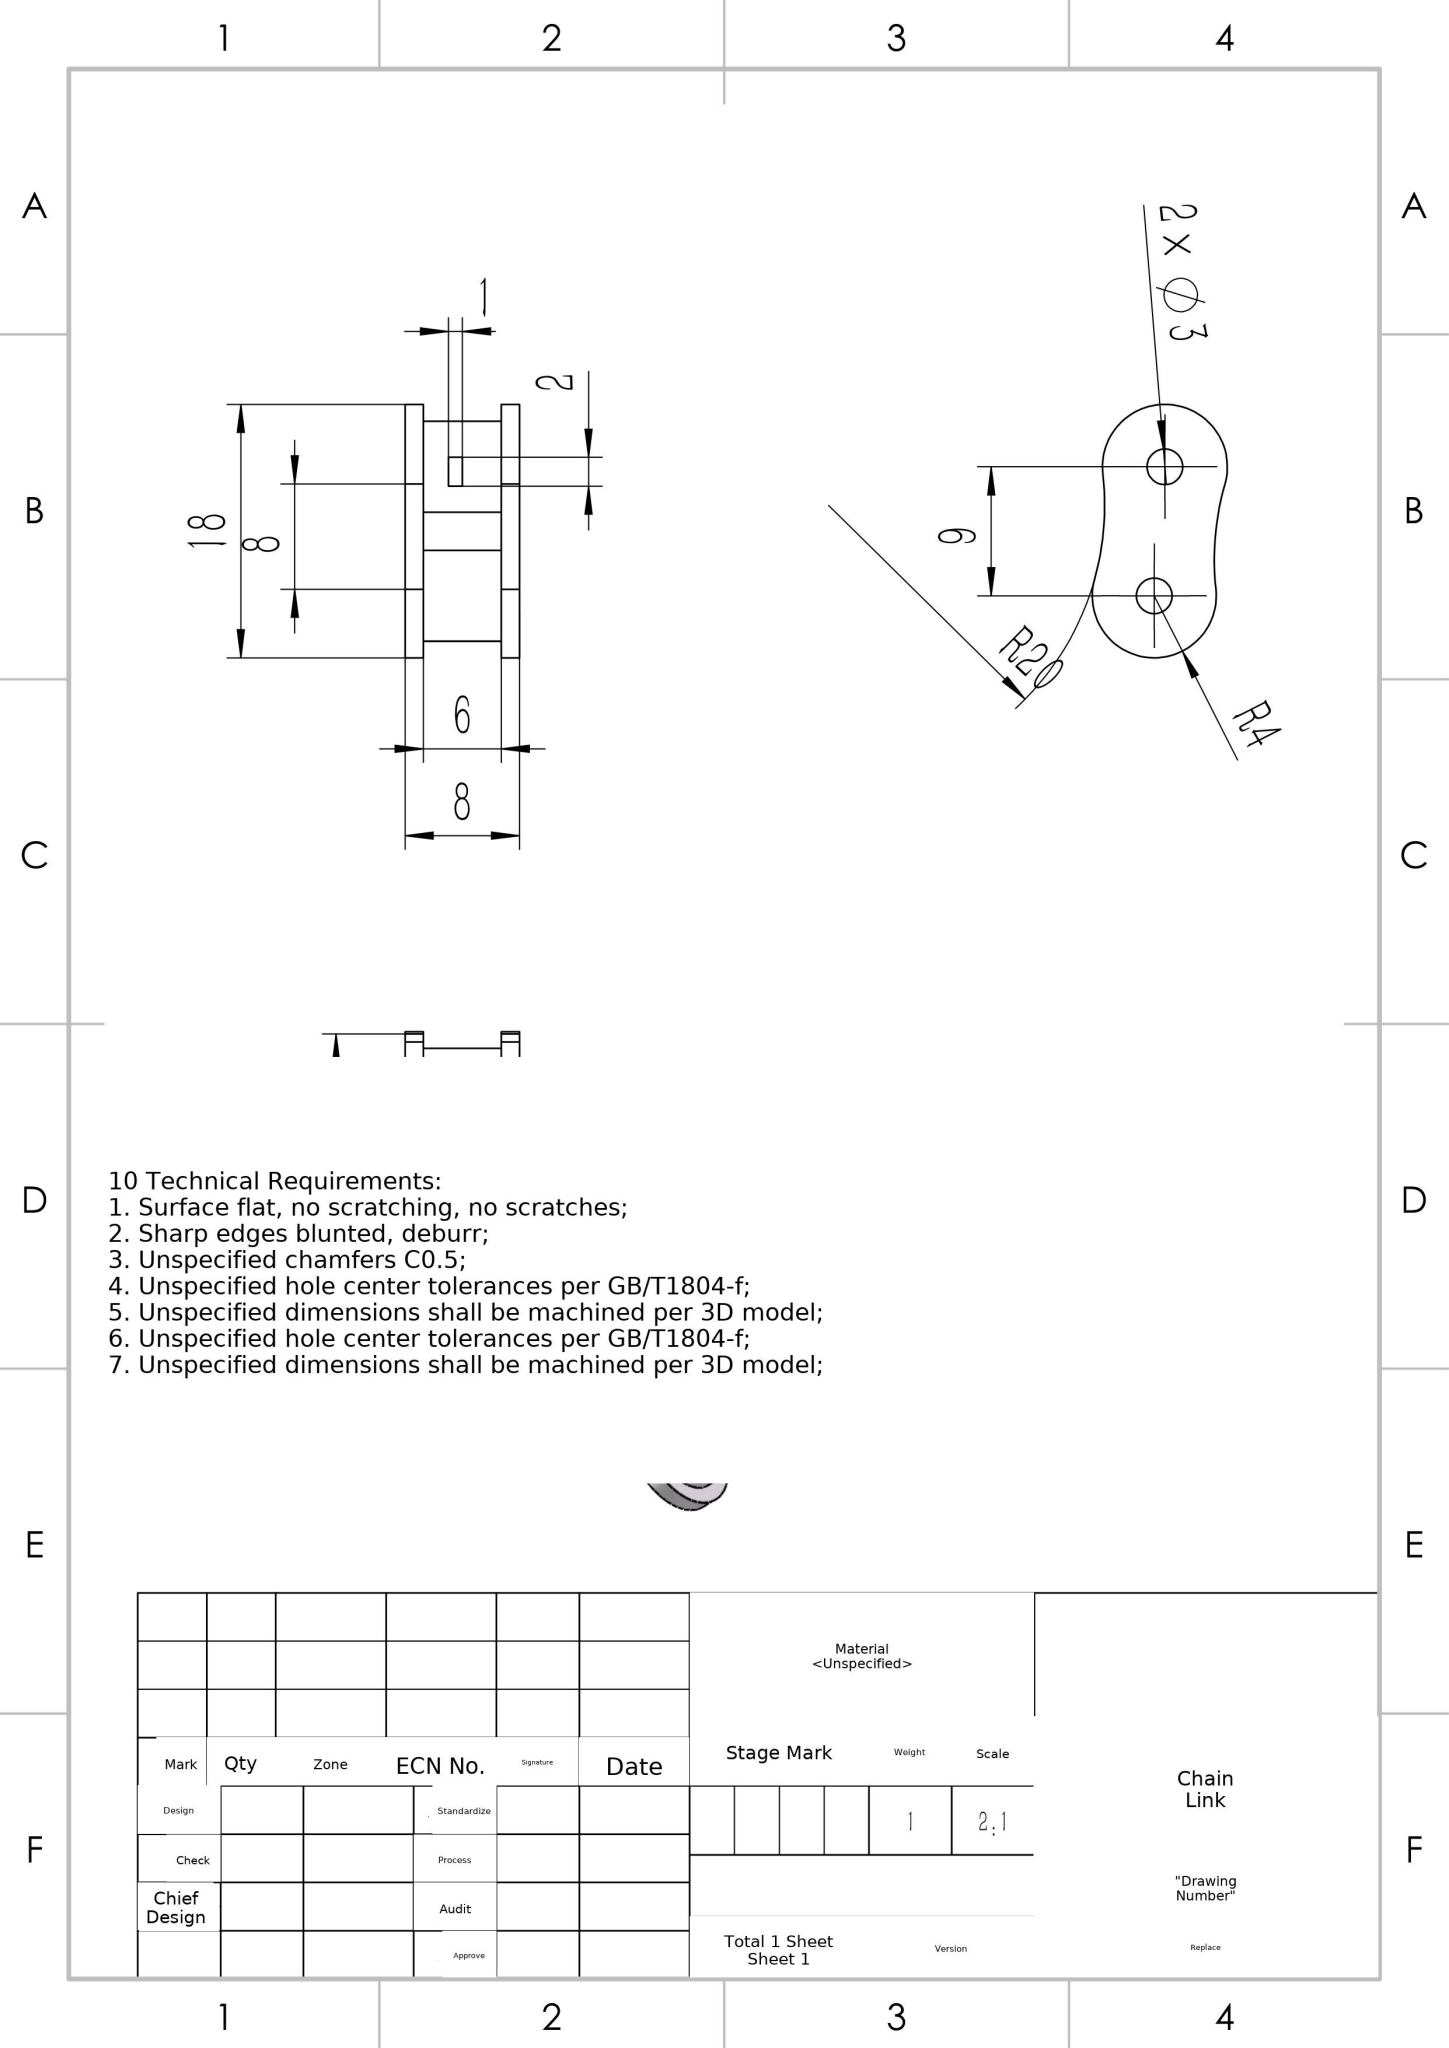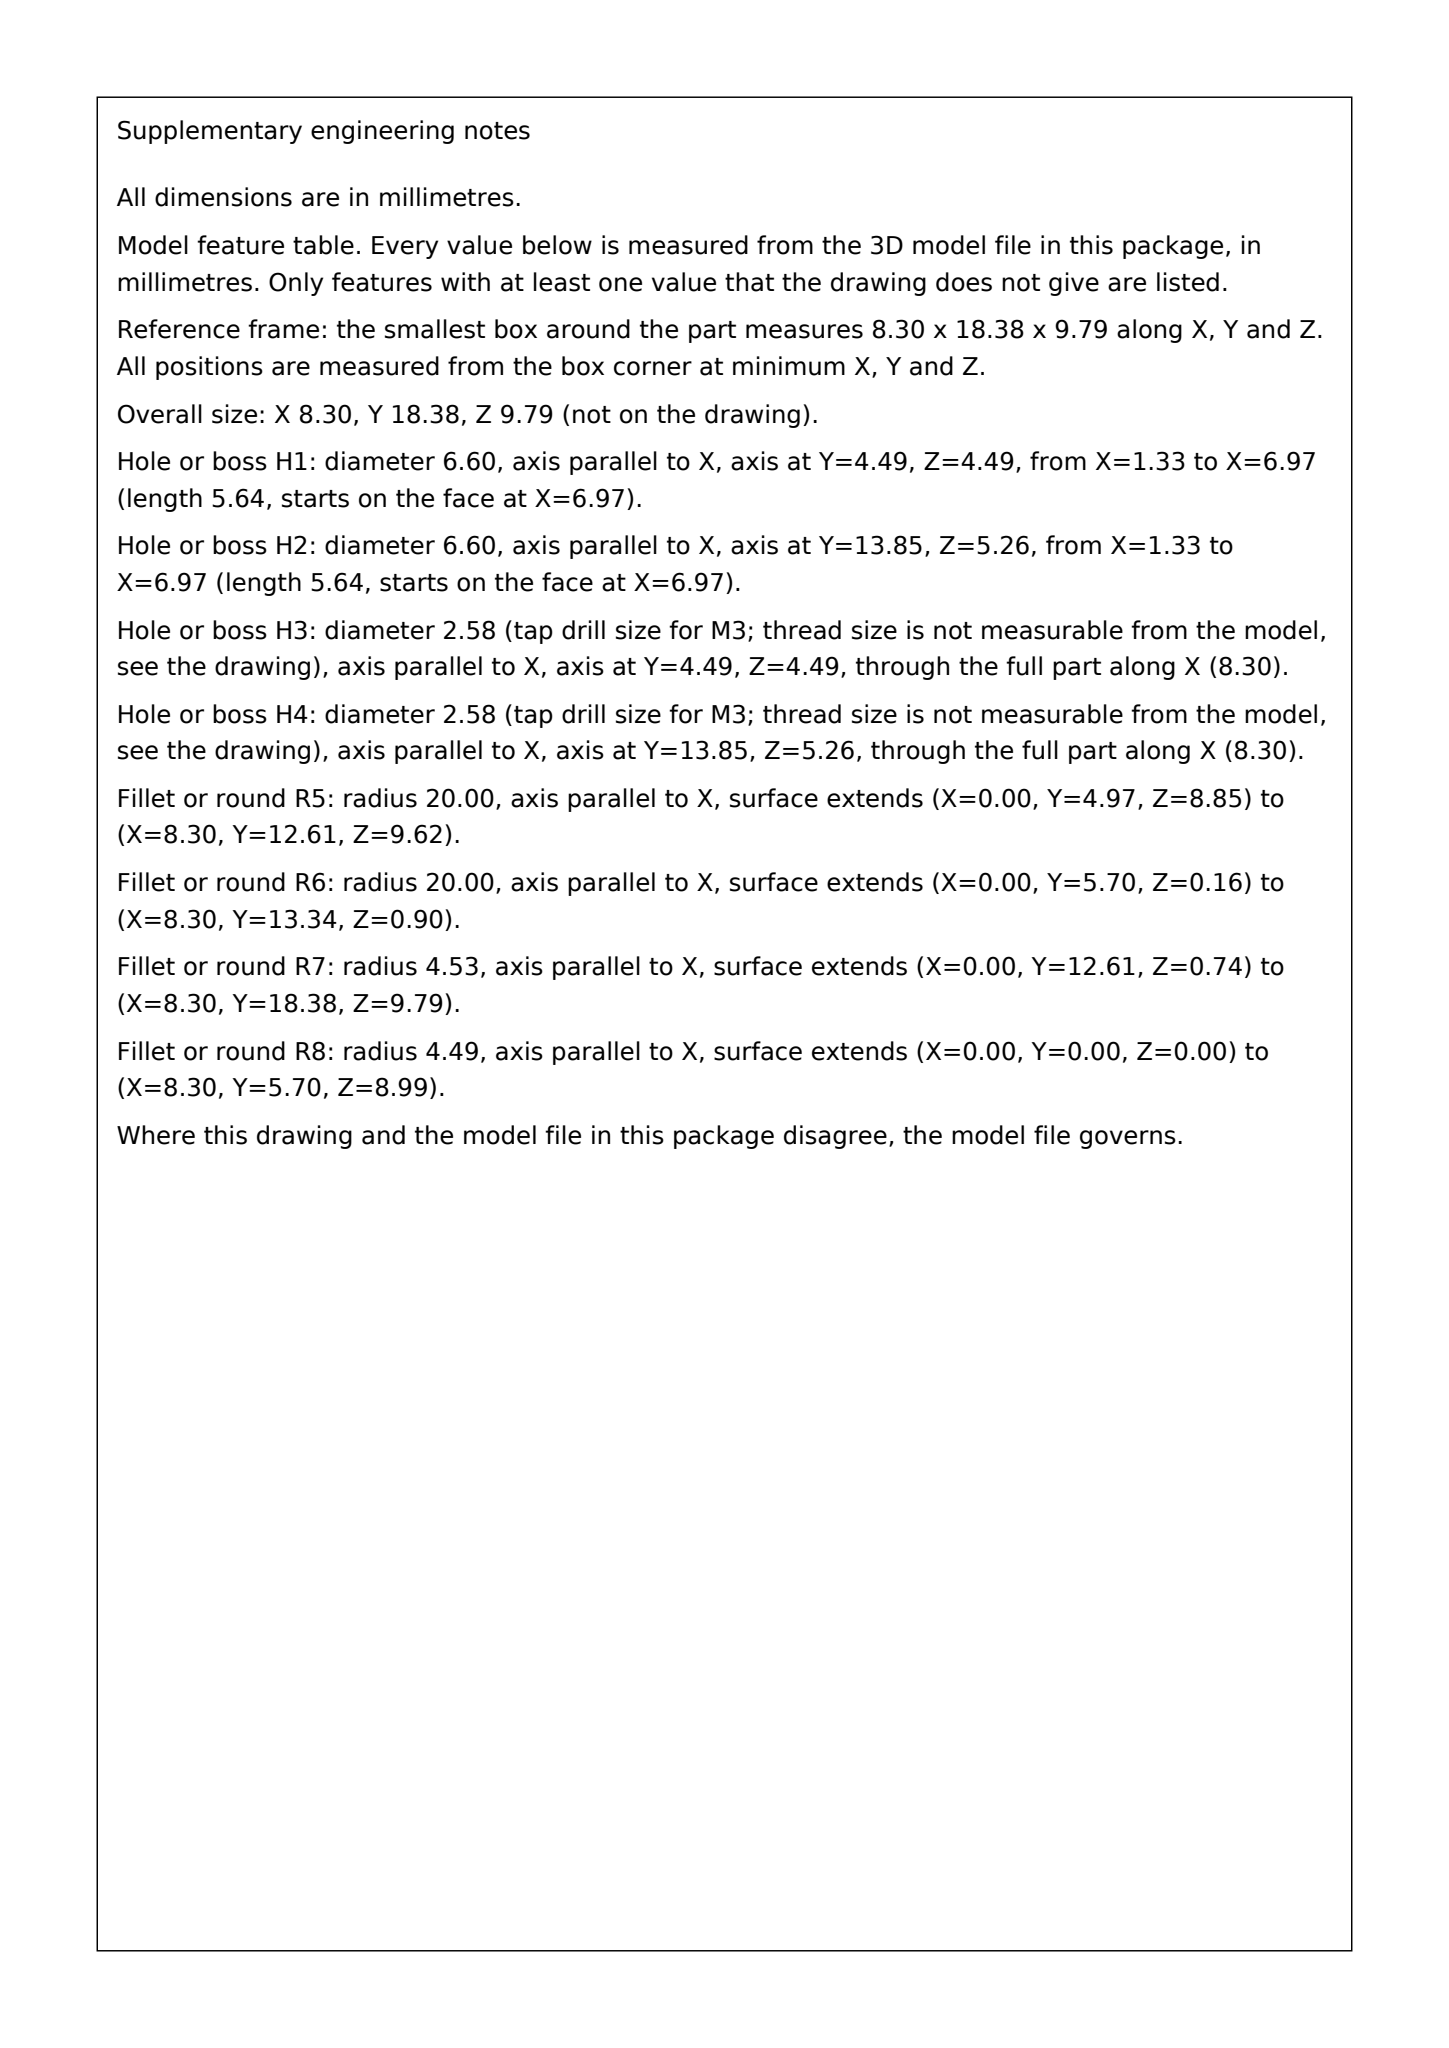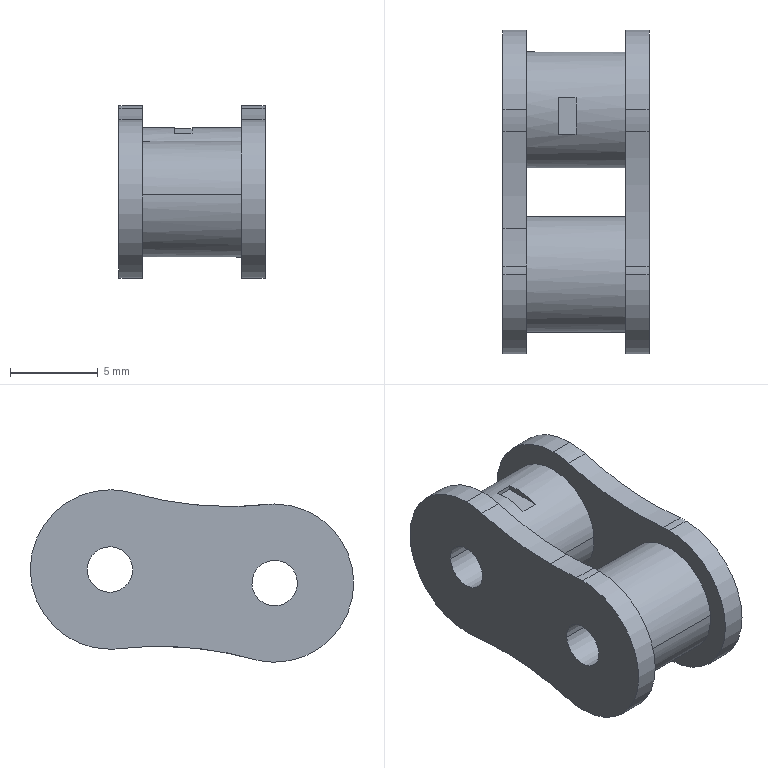Part | SolidWorks | mm | 1 solid | 34 faces | box 8.3 x 18.38 x 9.79 mm | volume 679 mm3 | cylinder 26 | plane 8 | commonest cylinder face diameters 9.054 x6 40 x6 8.987 x6 2.586 x4 6.59 x4